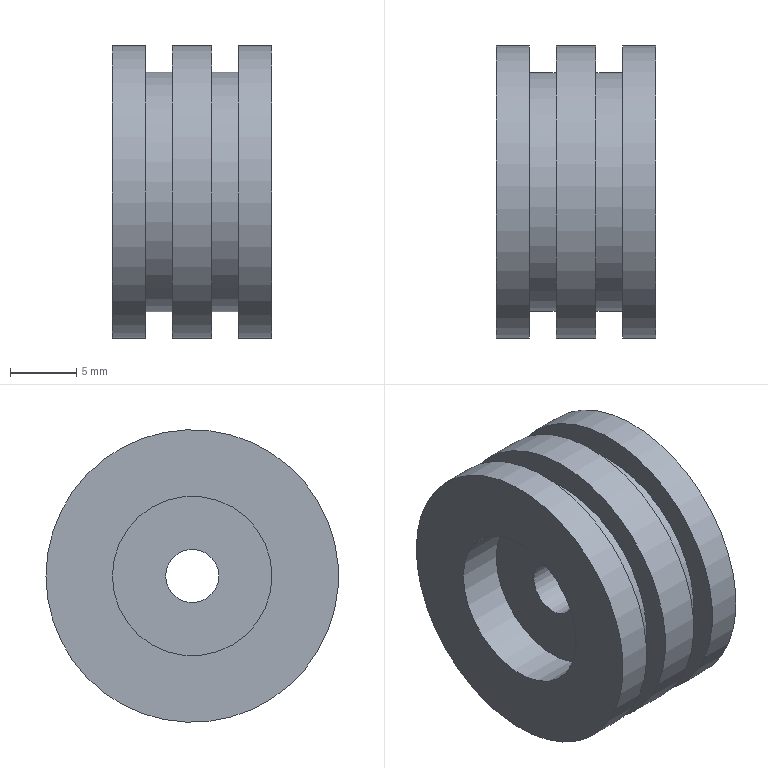Component | NX | PISTON | 1 solid | 16 faces | box 12 x 22 x 22 mm | volume 3525 mm3 | cylinder 8 | plane 8 | commonest cylinder face diameters 22 x3 18 x2 12 x1 6 x1 4 x1
STEP:
#1=CARTESIAN_POINT('',(0.,0.,0.));
#2=DIRECTION('',(0.,0.,1.));
#3=DIRECTION('',(1.,0.,0.));
#4=AXIS2_PLACEMENT_3D('',#1,#2,#3);
#5=CARTESIAN_POINT('',(-114.54,-11.,18.5));
#6=VERTEX_POINT('',#5);
#7=CARTESIAN_POINT('',(-114.54,-22.,18.5));
#8=DIRECTION('',(1.,0.,0.));
#9=DIRECTION('',(0.,1.,0.));
#10=AXIS2_PLACEMENT_3D('',#7,#8,#9);
#11=CIRCLE('',#10,11.);
#12=CARTESIAN_POINT('',(-110.04,-22.,18.5));
#13=DIRECTION('',(-1.,0.,0.));
#14=DIRECTION('',(0.,1.,0.));
#15=AXIS2_PLACEMENT_3D('',#12,#13,#14);
#16=CYLINDRICAL_SURFACE('',#15,11.);
#17=CARTESIAN_POINT('',(6.283,4.5));
#18=DIRECTION('',(-1.,0.));
#19=VECTOR('',#18,1.);
#20=LINE('',#17,#19);
#21=(GEOMETRIC_REPRESENTATION_CONTEXT(2)PARAMETRIC_REPRESENTATION_CONTEXT()REPRESENTATION_CONTEXT('',''));
#22=DEFINITIONAL_REPRESENTATION('',(#20),#21);
#23=PCURVE('',#16,#22);
#24=CARTESIAN_POINT('',(-114.54,-22.,18.5));
#25=DIRECTION('',(1.,0.,0.));
#26=DIRECTION('',(0.,-1.,0.));
#27=AXIS2_PLACEMENT_3D('',#24,#25,#26);
#28=PLANE('',#27);
#29=CARTESIAN_POINT('',(0.,0.));
#30=DIRECTION('',(-1.,0.));
#31=AXIS2_PLACEMENT_2D('',#29,#30);
#32=CIRCLE('',#31,11.);
#33=(GEOMETRIC_REPRESENTATION_CONTEXT(2)PARAMETRIC_REPRESENTATION_CONTEXT()REPRESENTATION_CONTEXT('',''));
#34=DEFINITIONAL_REPRESENTATION('',(#32),#33);
#35=PCURVE('',#28,#34);
#36=SURFACE_CURVE('',#11,(#23,#35),.PCURVE_S1.);
#37=EDGE_CURVE('',#6,#6,#36,.T.);
#38=ORIENTED_EDGE('',*,*,#37,.F.);
#39=CARTESIAN_POINT('',(-117.54,-11.,18.5));
#40=VERTEX_POINT('',#39);
#41=CARTESIAN_POINT('',(-114.54,-11.,18.5));
#42=CARTESIAN_POINT('',(-117.54,-11.,18.5));
#43=B_SPLINE_CURVE_WITH_KNOTS('',1,(#41,#42),.UNSPECIFIED.,.F.,.F.,(2,2),(4.5,7.5),.PIECEWISE_BEZIER_KNOTS.);
#44=CARTESIAN_POINT('',(6.283,0.));
#45=DIRECTION('',(0.,1.));
#46=VECTOR('',#45,1.);
#47=LINE('',#44,#46);
#48=(GEOMETRIC_REPRESENTATION_CONTEXT(2)PARAMETRIC_REPRESENTATION_CONTEXT()REPRESENTATION_CONTEXT('',''));
#49=DEFINITIONAL_REPRESENTATION('',(#47),#48);
#50=PCURVE('',#16,#49);
#51=CARTESIAN_POINT('',(0.,0.));
#52=DIRECTION('',(0.,1.));
#53=VECTOR('',#52,1.);
#54=LINE('',#51,#53);
#55=(GEOMETRIC_REPRESENTATION_CONTEXT(2)PARAMETRIC_REPRESENTATION_CONTEXT()REPRESENTATION_CONTEXT('',''));
#56=DEFINITIONAL_REPRESENTATION('',(#54),#55);
#57=PCURVE('',#16,#56);
#58=SEAM_CURVE('',#43,(#50,#57),.PCURVE_S1.);
#59=EDGE_CURVE('',#6,#40,#58,.T.);
#60=ORIENTED_EDGE('',*,*,#59,.T.);
#61=CARTESIAN_POINT('',(-117.54,-22.,18.5));
#62=DIRECTION('',(-1.,0.,0.));
#63=DIRECTION('',(0.,1.,0.));
#64=AXIS2_PLACEMENT_3D('',#61,#62,#63);
#65=CIRCLE('',#64,11.);
#66=CARTESIAN_POINT('',(0.,7.5));
#67=DIRECTION('',(1.,0.));
#68=VECTOR('',#67,1.);
#69=LINE('',#66,#68);
#70=(GEOMETRIC_REPRESENTATION_CONTEXT(2)PARAMETRIC_REPRESENTATION_CONTEXT()REPRESENTATION_CONTEXT('',''));
#71=DEFINITIONAL_REPRESENTATION('',(#69),#70);
#72=PCURVE('',#16,#71);
#73=CARTESIAN_POINT('',(-117.54,-22.,18.5));
#74=DIRECTION('',(-1.,0.,0.));
#75=DIRECTION('',(0.,1.,0.));
#76=AXIS2_PLACEMENT_3D('',#73,#74,#75);
#77=PLANE('',#76);
#78=CARTESIAN_POINT('',(0.,0.));
#79=DIRECTION('',(1.,0.));
#80=AXIS2_PLACEMENT_2D('',#78,#79);
#81=CIRCLE('',#80,11.);
#82=(GEOMETRIC_REPRESENTATION_CONTEXT(2)PARAMETRIC_REPRESENTATION_CONTEXT()REPRESENTATION_CONTEXT('',''));
#83=DEFINITIONAL_REPRESENTATION('',(#81),#82);
#84=PCURVE('',#77,#83);
#85=SURFACE_CURVE('',#65,(#72,#84),.PCURVE_S1.);
#86=EDGE_CURVE('',#40,#40,#85,.T.);
#87=ORIENTED_EDGE('',*,*,#86,.F.);
#88=ORIENTED_EDGE('',*,*,#59,.F.);
#89=EDGE_LOOP('',(#38,#60,#87,#88));
#90=FACE_BOUND('',#89,.T.);
#91=ADVANCED_FACE('',(#90),#16,.T.);
#92=CARTESIAN_POINT('',(-117.54,-13.,18.5));
#93=VERTEX_POINT('',#92);
#94=CARTESIAN_POINT('',(-117.54,-22.,18.5));
#95=DIRECTION('',(-1.,0.,0.));
#96=DIRECTION('',(0.,1.,0.));
#97=AXIS2_PLACEMENT_3D('',#94,#95,#96);
#98=CIRCLE('',#97,9.);
#99=CARTESIAN_POINT('',(-117.54,-22.,18.5));
#100=DIRECTION('',(-1.,0.,0.));
#101=DIRECTION('',(0.,1.,0.));
#102=AXIS2_PLACEMENT_3D('',#99,#100,#101);
#103=CYLINDRICAL_SURFACE('',#102,9.);
#104=CARTESIAN_POINT('',(0.,0.));
#105=DIRECTION('',(1.,0.));
#106=VECTOR('',#105,1.);
#107=LINE('',#104,#106);
#108=(GEOMETRIC_REPRESENTATION_CONTEXT(2)PARAMETRIC_REPRESENTATION_CONTEXT()REPRESENTATION_CONTEXT('',''));
#109=DEFINITIONAL_REPRESENTATION('',(#107),#108);
#110=PCURVE('',#103,#109);
#111=CARTESIAN_POINT('',(0.,0.));
#112=DIRECTION('',(1.,0.));
#113=AXIS2_PLACEMENT_2D('',#111,#112);
#114=CIRCLE('',#113,9.);
#115=(GEOMETRIC_REPRESENTATION_CONTEXT(2)PARAMETRIC_REPRESENTATION_CONTEXT()REPRESENTATION_CONTEXT('',''));
#116=DEFINITIONAL_REPRESENTATION('',(#114),#115);
#117=PCURVE('',#77,#116);
#118=SURFACE_CURVE('',#98,(#110,#117),.PCURVE_S1.);
#119=EDGE_CURVE('',#93,#93,#118,.T.);
#120=ORIENTED_EDGE('',*,*,#119,.T.);
#121=CARTESIAN_POINT('',(-119.54,-13.,18.5));
#122=VERTEX_POINT('',#121);
#123=CARTESIAN_POINT('',(-117.54,-13.,18.5));
#124=CARTESIAN_POINT('',(-119.54,-13.,18.5));
#125=B_SPLINE_CURVE_WITH_KNOTS('',1,(#123,#124),.UNSPECIFIED.,.F.,.F.,(2,2),(0.,2.),.PIECEWISE_BEZIER_KNOTS.);
#126=CARTESIAN_POINT('',(6.283,0.));
#127=DIRECTION('',(0.,1.));
#128=VECTOR('',#127,1.);
#129=LINE('',#126,#128);
#130=(GEOMETRIC_REPRESENTATION_CONTEXT(2)PARAMETRIC_REPRESENTATION_CONTEXT()REPRESENTATION_CONTEXT('',''));
#131=DEFINITIONAL_REPRESENTATION('',(#129),#130);
#132=PCURVE('',#103,#131);
#133=CARTESIAN_POINT('',(0.,0.));
#134=DIRECTION('',(0.,1.));
#135=VECTOR('',#134,1.);
#136=LINE('',#133,#135);
#137=(GEOMETRIC_REPRESENTATION_CONTEXT(2)PARAMETRIC_REPRESENTATION_CONTEXT()REPRESENTATION_CONTEXT('',''));
#138=DEFINITIONAL_REPRESENTATION('',(#136),#137);
#139=PCURVE('',#103,#138);
#140=SEAM_CURVE('',#125,(#132,#139),.PCURVE_S1.);
#141=EDGE_CURVE('',#93,#122,#140,.T.);
#142=ORIENTED_EDGE('',*,*,#141,.T.);
#143=CARTESIAN_POINT('',(-119.54,-22.,18.5));
#144=DIRECTION('',(-1.,0.,0.));
#145=DIRECTION('',(0.,1.,0.));
#146=AXIS2_PLACEMENT_3D('',#143,#144,#145);
#147=CIRCLE('',#146,9.);
#148=CARTESIAN_POINT('',(0.,2.));
#149=DIRECTION('',(1.,0.));
#150=VECTOR('',#149,1.);
#151=LINE('',#148,#150);
#152=(GEOMETRIC_REPRESENTATION_CONTEXT(2)PARAMETRIC_REPRESENTATION_CONTEXT()REPRESENTATION_CONTEXT('',''));
#153=DEFINITIONAL_REPRESENTATION('',(#151),#152);
#154=PCURVE('',#103,#153);
#155=CARTESIAN_POINT('',(-119.54,-22.,18.5));
#156=DIRECTION('',(-1.,0.,0.));
#157=DIRECTION('',(0.,1.,0.));
#158=AXIS2_PLACEMENT_3D('',#155,#156,#157);
#159=PLANE('',#158);
#160=CARTESIAN_POINT('',(0.,0.));
#161=DIRECTION('',(1.,0.));
#162=AXIS2_PLACEMENT_2D('',#160,#161);
#163=CIRCLE('',#162,9.);
#164=(GEOMETRIC_REPRESENTATION_CONTEXT(2)PARAMETRIC_REPRESENTATION_CONTEXT()REPRESENTATION_CONTEXT('',''));
#165=DEFINITIONAL_REPRESENTATION('',(#163),#164);
#166=PCURVE('',#159,#165);
#167=SURFACE_CURVE('',#147,(#154,#166),.PCURVE_S1.);
#168=EDGE_CURVE('',#122,#122,#167,.T.);
#169=ORIENTED_EDGE('',*,*,#168,.F.);
#170=ORIENTED_EDGE('',*,*,#141,.F.);
#171=EDGE_LOOP('',(#120,#142,#169,#170));
#172=FACE_BOUND('',#171,.T.);
#173=ADVANCED_FACE('',(#172),#103,.T.);
#174=ORIENTED_EDGE('',*,*,#86,.T.);
#175=EDGE_LOOP('',(#174));
#176=FACE_BOUND('',#175,.T.);
#177=ORIENTED_EDGE('',*,*,#119,.F.);
#178=EDGE_LOOP('',(#177));
#179=FACE_BOUND('',#178,.T.);
#180=ADVANCED_FACE('',(#176,#179),#77,.T.);
#181=CARTESIAN_POINT('',(-119.54,-11.,18.5));
#182=VERTEX_POINT('',#181);
#183=CARTESIAN_POINT('',(-119.54,-22.,18.5));
#184=DIRECTION('',(-1.,0.,0.));
#185=DIRECTION('',(0.,1.,0.));
#186=AXIS2_PLACEMENT_3D('',#183,#184,#185);
#187=CIRCLE('',#186,11.);
#188=CARTESIAN_POINT('',(0.,0.));
#189=DIRECTION('',(1.,0.));
#190=AXIS2_PLACEMENT_2D('',#188,#189);
#191=CIRCLE('',#190,11.);
#192=(GEOMETRIC_REPRESENTATION_CONTEXT(2)PARAMETRIC_REPRESENTATION_CONTEXT()REPRESENTATION_CONTEXT('',''));
#193=DEFINITIONAL_REPRESENTATION('',(#191),#192);
#194=PCURVE('',#159,#193);
#195=CARTESIAN_POINT('',(-110.04,-22.,18.5));
#196=DIRECTION('',(-1.,0.,0.));
#197=DIRECTION('',(0.,1.,0.));
#198=AXIS2_PLACEMENT_3D('',#195,#196,#197);
#199=CYLINDRICAL_SURFACE('',#198,11.);
#200=CARTESIAN_POINT('',(0.,9.5));
#201=DIRECTION('',(1.,0.));
#202=VECTOR('',#201,1.);
#203=LINE('',#200,#202);
#204=(GEOMETRIC_REPRESENTATION_CONTEXT(2)PARAMETRIC_REPRESENTATION_CONTEXT()REPRESENTATION_CONTEXT('',''));
#205=DEFINITIONAL_REPRESENTATION('',(#203),#204);
#206=PCURVE('',#199,#205);
#207=SURFACE_CURVE('',#187,(#194,#206),.PCURVE_S1.);
#208=EDGE_CURVE('',#182,#182,#207,.T.);
#209=ORIENTED_EDGE('',*,*,#208,.F.);
#210=EDGE_LOOP('',(#209));
#211=FACE_BOUND('',#210,.T.);
#212=ORIENTED_EDGE('',*,*,#168,.T.);
#213=EDGE_LOOP('',(#212));
#214=FACE_BOUND('',#213,.T.);
#215=ADVANCED_FACE('',(#211,#214),#159,.F.);
#216=CARTESIAN_POINT('',(-122.04,-16.,18.5));
#217=VERTEX_POINT('',#216);
#218=CARTESIAN_POINT('',(-122.04,-22.,18.5));
#219=DIRECTION('',(1.,0.,0.));
#220=DIRECTION('',(0.,1.,0.));
#221=AXIS2_PLACEMENT_3D('',#218,#219,#220);
#222=CIRCLE('',#221,6.);
#223=CARTESIAN_POINT('',(-122.04,-22.,18.5));
#224=DIRECTION('',(-1.,0.,0.));
#225=DIRECTION('',(0.,1.,0.));
#226=AXIS2_PLACEMENT_3D('',#223,#224,#225);
#227=PLANE('',#226);
#228=CARTESIAN_POINT('',(6.,0.));
#229=CARTESIAN_POINT('',(6.,-10.392));
#230=CARTESIAN_POINT('',(-3.,-5.196));
#231=CARTESIAN_POINT('',(-12.,-0.));
#232=CARTESIAN_POINT('',(-3.,5.196));
#233=CARTESIAN_POINT('',(6.,10.392));
#234=CARTESIAN_POINT('',(6.,0.));
#235=(BOUNDED_CURVE()B_SPLINE_CURVE(2,(#228,#229,#230,#231,#232,#233,#234),.UNSPECIFIED.,.T.,.F.)B_SPLINE_CURVE_WITH_KNOTS((1,2,2,2,2,1),(-2.094,0.,2.094,4.189,6.283,8.378),.UNSPECIFIED.)CURVE()GEOMETRIC_REPRESENTATION_ITEM()RATIONAL_B_SPLINE_CURVE((1.,0.5,1.,0.5,1.,0.5,1.))REPRESENTATION_ITEM(''));
#236=(GEOMETRIC_REPRESENTATION_CONTEXT(2)PARAMETRIC_REPRESENTATION_CONTEXT()REPRESENTATION_CONTEXT('',''));
#237=DEFINITIONAL_REPRESENTATION('',(#235),#236);
#238=PCURVE('',#227,#237);
#239=CARTESIAN_POINT('',(-118.54,-22.,18.5));
#240=DIRECTION('',(-1.,0.,0.));
#241=DIRECTION('',(0.,1.,0.));
#242=AXIS2_PLACEMENT_3D('',#239,#240,#241);
#243=CYLINDRICAL_SURFACE('',#242,6.);
#244=CARTESIAN_POINT('',(6.283,3.5));
#245=DIRECTION('',(-1.,0.));
#246=VECTOR('',#245,1.);
#247=LINE('',#244,#246);
#248=(GEOMETRIC_REPRESENTATION_CONTEXT(2)PARAMETRIC_REPRESENTATION_CONTEXT()REPRESENTATION_CONTEXT('',''));
#249=DEFINITIONAL_REPRESENTATION('',(#247),#248);
#250=PCURVE('',#243,#249);
#251=SURFACE_CURVE('',#222,(#238,#250),.PCURVE_S1.);
#252=EDGE_CURVE('',#217,#217,#251,.T.);
#253=ORIENTED_EDGE('',*,*,#252,.T.);
#254=EDGE_LOOP('',(#253));
#255=FACE_BOUND('',#254,.T.);
#256=CARTESIAN_POINT('',(-122.04,-11.,18.5));
#257=VERTEX_POINT('',#256);
#258=CARTESIAN_POINT('',(-122.04,-22.,18.5));
#259=DIRECTION('',(1.,0.,0.));
#260=DIRECTION('',(0.,1.,0.));
#261=AXIS2_PLACEMENT_3D('',#258,#259,#260);
#262=CIRCLE('',#261,11.);
#263=CARTESIAN_POINT('',(11.,0.));
#264=CARTESIAN_POINT('',(11.,-19.053));
#265=CARTESIAN_POINT('',(-5.5,-9.526));
#266=CARTESIAN_POINT('',(-22.,-0.));
#267=CARTESIAN_POINT('',(-5.5,9.526));
#268=CARTESIAN_POINT('',(11.,19.053));
#269=CARTESIAN_POINT('',(11.,0.));
#270=(BOUNDED_CURVE()B_SPLINE_CURVE(2,(#263,#264,#265,#266,#267,#268,#269),.UNSPECIFIED.,.T.,.F.)B_SPLINE_CURVE_WITH_KNOTS((1,2,2,2,2,1),(-2.094,0.,2.094,4.189,6.283,8.378),.UNSPECIFIED.)CURVE()GEOMETRIC_REPRESENTATION_ITEM()RATIONAL_B_SPLINE_CURVE((1.,0.5,1.,0.5,1.,0.5,1.))REPRESENTATION_ITEM(''));
#271=(GEOMETRIC_REPRESENTATION_CONTEXT(2)PARAMETRIC_REPRESENTATION_CONTEXT()REPRESENTATION_CONTEXT('',''));
#272=DEFINITIONAL_REPRESENTATION('',(#270),#271);
#273=PCURVE('',#227,#272);
#274=CARTESIAN_POINT('',(6.283,12.));
#275=DIRECTION('',(-1.,0.));
#276=VECTOR('',#275,1.);
#277=LINE('',#274,#276);
#278=(GEOMETRIC_REPRESENTATION_CONTEXT(2)PARAMETRIC_REPRESENTATION_CONTEXT()REPRESENTATION_CONTEXT('',''));
#279=DEFINITIONAL_REPRESENTATION('',(#277),#278);
#280=PCURVE('',#199,#279);
#281=SURFACE_CURVE('',#262,(#273,#280),.PCURVE_S1.);
#282=EDGE_CURVE('',#257,#257,#281,.T.);
#283=ORIENTED_EDGE('',*,*,#282,.F.);
#284=EDGE_LOOP('',(#283));
#285=FACE_BOUND('',#284,.T.);
#286=ADVANCED_FACE('',(#255,#285),#227,.T.);
#287=ORIENTED_EDGE('',*,*,#282,.T.);
#288=CARTESIAN_POINT('',(-119.54,-11.,18.5));
#289=CARTESIAN_POINT('',(-122.04,-11.,18.5));
#290=B_SPLINE_CURVE_WITH_KNOTS('',1,(#288,#289),.UNSPECIFIED.,.F.,.F.,(2,2),(9.5,12.),.PIECEWISE_BEZIER_KNOTS.);
#291=CARTESIAN_POINT('',(0.,0.));
#292=DIRECTION('',(0.,1.));
#293=VECTOR('',#292,1.);
#294=LINE('',#291,#293);
#295=(GEOMETRIC_REPRESENTATION_CONTEXT(2)PARAMETRIC_REPRESENTATION_CONTEXT()REPRESENTATION_CONTEXT('',''));
#296=DEFINITIONAL_REPRESENTATION('',(#294),#295);
#297=PCURVE('',#199,#296);
#298=CARTESIAN_POINT('',(6.283,0.));
#299=DIRECTION('',(0.,1.));
#300=VECTOR('',#299,1.);
#301=LINE('',#298,#300);
#302=(GEOMETRIC_REPRESENTATION_CONTEXT(2)PARAMETRIC_REPRESENTATION_CONTEXT()REPRESENTATION_CONTEXT('',''));
#303=DEFINITIONAL_REPRESENTATION('',(#301),#302);
#304=PCURVE('',#199,#303);
#305=SEAM_CURVE('',#290,(#297,#304),.PCURVE_S1.);
#306=EDGE_CURVE('',#182,#257,#305,.T.);
#307=ORIENTED_EDGE('',*,*,#306,.F.);
#308=ORIENTED_EDGE('',*,*,#208,.T.);
#309=ORIENTED_EDGE('',*,*,#306,.T.);
#310=EDGE_LOOP('',(#287,#307,#308,#309));
#311=FACE_BOUND('',#310,.T.);
#312=ADVANCED_FACE('',(#311),#199,.T.);
#313=CARTESIAN_POINT('',(-114.54,-13.,18.5));
#314=VERTEX_POINT('',#313);
#315=CARTESIAN_POINT('',(-114.54,-22.,18.5));
#316=DIRECTION('',(1.,0.,0.));
#317=DIRECTION('',(0.,1.,0.));
#318=AXIS2_PLACEMENT_3D('',#315,#316,#317);
#319=CIRCLE('',#318,9.);
#320=CARTESIAN_POINT('',(-114.54,-22.,18.5));
#321=DIRECTION('',(1.,0.,0.));
#322=DIRECTION('',(0.,-1.,0.));
#323=AXIS2_PLACEMENT_3D('',#320,#321,#322);
#324=CYLINDRICAL_SURFACE('',#323,9.);
#325=CARTESIAN_POINT('',(3.142,0.));
#326=DIRECTION('',(1.,0.));
#327=VECTOR('',#326,1.);
#328=LINE('',#325,#327);
#329=(GEOMETRIC_REPRESENTATION_CONTEXT(2)PARAMETRIC_REPRESENTATION_CONTEXT()REPRESENTATION_CONTEXT('',''));
#330=DEFINITIONAL_REPRESENTATION('',(#328),#329);
#331=PCURVE('',#324,#330);
#332=CARTESIAN_POINT('',(0.,0.));
#333=DIRECTION('',(-1.,0.));
#334=AXIS2_PLACEMENT_2D('',#332,#333);
#335=CIRCLE('',#334,9.);
#336=(GEOMETRIC_REPRESENTATION_CONTEXT(2)PARAMETRIC_REPRESENTATION_CONTEXT()REPRESENTATION_CONTEXT('',''));
#337=DEFINITIONAL_REPRESENTATION('',(#335),#336);
#338=PCURVE('',#28,#337);
#339=SURFACE_CURVE('',#319,(#331,#338),.PCURVE_S1.);
#340=EDGE_CURVE('',#314,#314,#339,.T.);
#341=ORIENTED_EDGE('',*,*,#340,.T.);
#342=CARTESIAN_POINT('',(-112.54,-13.,18.5));
#343=VERTEX_POINT('',#342);
#344=CARTESIAN_POINT('',(-114.54,-13.,18.5));
#345=CARTESIAN_POINT('',(-112.54,-13.,18.5));
#346=B_SPLINE_CURVE_WITH_KNOTS('',1,(#344,#345),.UNSPECIFIED.,.F.,.F.,(2,2),(0.,2.),.PIECEWISE_BEZIER_KNOTS.);
#347=CARTESIAN_POINT('',(9.425,0.));
#348=DIRECTION('',(0.,1.));
#349=VECTOR('',#348,1.);
#350=LINE('',#347,#349);
#351=(GEOMETRIC_REPRESENTATION_CONTEXT(2)PARAMETRIC_REPRESENTATION_CONTEXT()REPRESENTATION_CONTEXT('',''));
#352=DEFINITIONAL_REPRESENTATION('',(#350),#351);
#353=PCURVE('',#324,#352);
#354=CARTESIAN_POINT('',(3.142,0.));
#355=DIRECTION('',(0.,1.));
#356=VECTOR('',#355,1.);
#357=LINE('',#354,#356);
#358=(GEOMETRIC_REPRESENTATION_CONTEXT(2)PARAMETRIC_REPRESENTATION_CONTEXT()REPRESENTATION_CONTEXT('',''));
#359=DEFINITIONAL_REPRESENTATION('',(#357),#358);
#360=PCURVE('',#324,#359);
#361=SEAM_CURVE('',#346,(#353,#360),.PCURVE_S1.);
#362=EDGE_CURVE('',#314,#343,#361,.T.);
#363=ORIENTED_EDGE('',*,*,#362,.T.);
#364=CARTESIAN_POINT('',(-112.54,-22.,18.5));
#365=DIRECTION('',(1.,0.,0.));
#366=DIRECTION('',(0.,1.,0.));
#367=AXIS2_PLACEMENT_3D('',#364,#365,#366);
#368=CIRCLE('',#367,9.);
#369=CARTESIAN_POINT('',(3.142,2.));
#370=DIRECTION('',(1.,0.));
#371=VECTOR('',#370,1.);
#372=LINE('',#369,#371);
#373=(GEOMETRIC_REPRESENTATION_CONTEXT(2)PARAMETRIC_REPRESENTATION_CONTEXT()REPRESENTATION_CONTEXT('',''));
#374=DEFINITIONAL_REPRESENTATION('',(#372),#373);
#375=PCURVE('',#324,#374);
#376=CARTESIAN_POINT('',(-112.54,-22.,18.5));
#377=DIRECTION('',(1.,0.,0.));
#378=DIRECTION('',(0.,-1.,0.));
#379=AXIS2_PLACEMENT_3D('',#376,#377,#378);
#380=PLANE('',#379);
#381=CARTESIAN_POINT('',(0.,0.));
#382=DIRECTION('',(-1.,0.));
#383=AXIS2_PLACEMENT_2D('',#381,#382);
#384=CIRCLE('',#383,9.);
#385=(GEOMETRIC_REPRESENTATION_CONTEXT(2)PARAMETRIC_REPRESENTATION_CONTEXT()REPRESENTATION_CONTEXT('',''));
#386=DEFINITIONAL_REPRESENTATION('',(#384),#385);
#387=PCURVE('',#380,#386);
#388=SURFACE_CURVE('',#368,(#375,#387),.PCURVE_S1.);
#389=EDGE_CURVE('',#343,#343,#388,.T.);
#390=ORIENTED_EDGE('',*,*,#389,.F.);
#391=ORIENTED_EDGE('',*,*,#362,.F.);
#392=EDGE_LOOP('',(#341,#363,#390,#391));
#393=FACE_BOUND('',#392,.T.);
#394=ADVANCED_FACE('',(#393),#324,.T.);
#395=ORIENTED_EDGE('',*,*,#37,.T.);
#396=EDGE_LOOP('',(#395));
#397=FACE_BOUND('',#396,.T.);
#398=ORIENTED_EDGE('',*,*,#340,.F.);
#399=EDGE_LOOP('',(#398));
#400=FACE_BOUND('',#399,.T.);
#401=ADVANCED_FACE('',(#397,#400),#28,.T.);
#402=CARTESIAN_POINT('',(-112.54,-11.,18.5));
#403=VERTEX_POINT('',#402);
#404=CARTESIAN_POINT('',(-112.54,-22.,18.5));
#405=DIRECTION('',(1.,0.,0.));
#406=DIRECTION('',(0.,1.,0.));
#407=AXIS2_PLACEMENT_3D('',#404,#405,#406);
#408=CIRCLE('',#407,11.);
#409=CARTESIAN_POINT('',(0.,0.));
#410=DIRECTION('',(-1.,0.));
#411=AXIS2_PLACEMENT_2D('',#409,#410);
#412=CIRCLE('',#411,11.);
#413=(GEOMETRIC_REPRESENTATION_CONTEXT(2)PARAMETRIC_REPRESENTATION_CONTEXT()REPRESENTATION_CONTEXT('',''));
#414=DEFINITIONAL_REPRESENTATION('',(#412),#413);
#415=PCURVE('',#380,#414);
#416=CARTESIAN_POINT('',(-110.04,-22.,18.5));
#417=DIRECTION('',(-1.,0.,0.));
#418=DIRECTION('',(0.,1.,0.));
#419=AXIS2_PLACEMENT_3D('',#416,#417,#418);
#420=CYLINDRICAL_SURFACE('',#419,11.);
#421=CARTESIAN_POINT('',(6.283,2.5));
#422=DIRECTION('',(-1.,0.));
#423=VECTOR('',#422,1.);
#424=LINE('',#421,#423);
#425=(GEOMETRIC_REPRESENTATION_CONTEXT(2)PARAMETRIC_REPRESENTATION_CONTEXT()REPRESENTATION_CONTEXT('',''));
#426=DEFINITIONAL_REPRESENTATION('',(#424),#425);
#427=PCURVE('',#420,#426);
#428=SURFACE_CURVE('',#408,(#415,#427),.PCURVE_S1.);
#429=EDGE_CURVE('',#403,#403,#428,.T.);
#430=ORIENTED_EDGE('',*,*,#429,.F.);
#431=EDGE_LOOP('',(#430));
#432=FACE_BOUND('',#431,.T.);
#433=ORIENTED_EDGE('',*,*,#389,.T.);
#434=EDGE_LOOP('',(#433));
#435=FACE_BOUND('',#434,.T.);
#436=ADVANCED_FACE('',(#432,#435),#380,.F.);
#437=CARTESIAN_POINT('',(-110.04,-19.,18.5));
#438=VERTEX_POINT('',#437);
#439=CARTESIAN_POINT('',(-110.04,-22.,18.5));
#440=DIRECTION('',(-1.,0.,0.));
#441=DIRECTION('',(0.,1.,0.));
#442=AXIS2_PLACEMENT_3D('',#439,#440,#441);
#443=CIRCLE('',#442,3.);
#444=CARTESIAN_POINT('',(-110.04,-22.,18.5));
#445=DIRECTION('',(1.,0.,0.));
#446=DIRECTION('',(0.,-1.,0.));
#447=AXIS2_PLACEMENT_3D('',#444,#445,#446);
#448=PLANE('',#447);
#449=CARTESIAN_POINT('',(-3.,0.));
#450=CARTESIAN_POINT('',(-3.,5.196));
#451=CARTESIAN_POINT('',(1.5,2.598));
#452=CARTESIAN_POINT('',(6.,0.));
#453=CARTESIAN_POINT('',(1.5,-2.598));
#454=CARTESIAN_POINT('',(-3.,-5.196));
#455=CARTESIAN_POINT('',(-3.,0.));
#456=(BOUNDED_CURVE()B_SPLINE_CURVE(2,(#449,#450,#451,#452,#453,#454,#455),.UNSPECIFIED.,.T.,.F.)B_SPLINE_CURVE_WITH_KNOTS((1,2,2,2,2,1),(-2.094,0.,2.094,4.189,6.283,8.378),.UNSPECIFIED.)CURVE()GEOMETRIC_REPRESENTATION_ITEM()RATIONAL_B_SPLINE_CURVE((1.,0.5,1.,0.5,1.,0.5,1.))REPRESENTATION_ITEM(''));
#457=(GEOMETRIC_REPRESENTATION_CONTEXT(2)PARAMETRIC_REPRESENTATION_CONTEXT()REPRESENTATION_CONTEXT('',''));
#458=DEFINITIONAL_REPRESENTATION('',(#456),#457);
#459=PCURVE('',#448,#458);
#460=CARTESIAN_POINT('',(-112.04,-22.,18.5));
#461=DIRECTION('',(1.,0.,0.));
#462=DIRECTION('',(0.,-1.,0.));
#463=AXIS2_PLACEMENT_3D('',#460,#461,#462);
#464=CYLINDRICAL_SURFACE('',#463,3.);
#465=CARTESIAN_POINT('',(9.425,2.));
#466=DIRECTION('',(-1.,0.));
#467=VECTOR('',#466,1.);
#468=LINE('',#465,#467);
#469=(GEOMETRIC_REPRESENTATION_CONTEXT(2)PARAMETRIC_REPRESENTATION_CONTEXT()REPRESENTATION_CONTEXT('',''));
#470=DEFINITIONAL_REPRESENTATION('',(#468),#469);
#471=PCURVE('',#464,#470);
#472=SURFACE_CURVE('',#443,(#459,#471),.PCURVE_S1.);
#473=EDGE_CURVE('',#438,#438,#472,.T.);
#474=ORIENTED_EDGE('',*,*,#473,.T.);
#475=EDGE_LOOP('',(#474));
#476=FACE_BOUND('',#475,.T.);
#477=CARTESIAN_POINT('',(-110.04,-11.,18.5));
#478=VERTEX_POINT('',#477);
#479=CARTESIAN_POINT('',(-110.04,-22.,18.5));
#480=DIRECTION('',(-1.,0.,0.));
#481=DIRECTION('',(0.,1.,0.));
#482=AXIS2_PLACEMENT_3D('',#479,#480,#481);
#483=CIRCLE('',#482,11.);
#484=CARTESIAN_POINT('',(-11.,0.));
#485=CARTESIAN_POINT('',(-11.,19.053));
#486=CARTESIAN_POINT('',(5.5,9.526));
#487=CARTESIAN_POINT('',(22.,0.));
#488=CARTESIAN_POINT('',(5.5,-9.526));
#489=CARTESIAN_POINT('',(-11.,-19.053));
#490=CARTESIAN_POINT('',(-11.,0.));
#491=(BOUNDED_CURVE()B_SPLINE_CURVE(2,(#484,#485,#486,#487,#488,#489,#490),.UNSPECIFIED.,.T.,.F.)B_SPLINE_CURVE_WITH_KNOTS((1,2,2,2,2,1),(-2.094,0.,2.094,4.189,6.283,8.378),.UNSPECIFIED.)CURVE()GEOMETRIC_REPRESENTATION_ITEM()RATIONAL_B_SPLINE_CURVE((1.,0.5,1.,0.5,1.,0.5,1.))REPRESENTATION_ITEM(''));
#492=(GEOMETRIC_REPRESENTATION_CONTEXT(2)PARAMETRIC_REPRESENTATION_CONTEXT()REPRESENTATION_CONTEXT('',''));
#493=DEFINITIONAL_REPRESENTATION('',(#491),#492);
#494=PCURVE('',#448,#493);
#495=CARTESIAN_POINT('',(0.,0.));
#496=DIRECTION('',(1.,0.));
#497=VECTOR('',#496,1.);
#498=LINE('',#495,#497);
#499=(GEOMETRIC_REPRESENTATION_CONTEXT(2)PARAMETRIC_REPRESENTATION_CONTEXT()REPRESENTATION_CONTEXT('',''));
#500=DEFINITIONAL_REPRESENTATION('',(#498),#499);
#501=PCURVE('',#420,#500);
#502=SURFACE_CURVE('',#483,(#494,#501),.PCURVE_S1.);
#503=EDGE_CURVE('',#478,#478,#502,.T.);
#504=ORIENTED_EDGE('',*,*,#503,.F.);
#505=EDGE_LOOP('',(#504));
#506=FACE_BOUND('',#505,.T.);
#507=ADVANCED_FACE('',(#476,#506),#448,.T.);
#508=ORIENTED_EDGE('',*,*,#503,.T.);
#509=CARTESIAN_POINT('',(-110.04,-11.,18.5));
#510=CARTESIAN_POINT('',(-112.54,-11.,18.5));
#511=B_SPLINE_CURVE_WITH_KNOTS('',1,(#509,#510),.UNSPECIFIED.,.F.,.F.,(2,2),(0.,2.5),.PIECEWISE_BEZIER_KNOTS.);
#512=CARTESIAN_POINT('',(6.283,0.));
#513=DIRECTION('',(0.,1.));
#514=VECTOR('',#513,1.);
#515=LINE('',#512,#514);
#516=(GEOMETRIC_REPRESENTATION_CONTEXT(2)PARAMETRIC_REPRESENTATION_CONTEXT()REPRESENTATION_CONTEXT('',''));
#517=DEFINITIONAL_REPRESENTATION('',(#515),#516);
#518=PCURVE('',#420,#517);
#519=CARTESIAN_POINT('',(0.,0.));
#520=DIRECTION('',(0.,1.));
#521=VECTOR('',#520,1.);
#522=LINE('',#519,#521);
#523=(GEOMETRIC_REPRESENTATION_CONTEXT(2)PARAMETRIC_REPRESENTATION_CONTEXT()REPRESENTATION_CONTEXT('',''));
#524=DEFINITIONAL_REPRESENTATION('',(#522),#523);
#525=PCURVE('',#420,#524);
#526=SEAM_CURVE('',#511,(#518,#525),.PCURVE_S1.);
#527=EDGE_CURVE('',#478,#403,#526,.T.);
#528=ORIENTED_EDGE('',*,*,#527,.T.);
#529=ORIENTED_EDGE('',*,*,#429,.T.);
#530=ORIENTED_EDGE('',*,*,#527,.F.);
#531=EDGE_LOOP('',(#508,#528,#529,#530));
#532=FACE_BOUND('',#531,.T.);
#533=ADVANCED_FACE('',(#532),#420,.T.);
#534=CARTESIAN_POINT('',(-118.54,-16.,18.5));
#535=VERTEX_POINT('',#534);
#536=CARTESIAN_POINT('',(-118.54,-22.,18.5));
#537=DIRECTION('',(-1.,0.,0.));
#538=DIRECTION('',(0.,1.,0.));
#539=AXIS2_PLACEMENT_3D('',#536,#537,#538);
#540=CIRCLE('',#539,6.);
#541=CARTESIAN_POINT('',(0.,0.));
#542=DIRECTION('',(1.,0.));
#543=VECTOR('',#542,1.);
#544=LINE('',#541,#543);
#545=(GEOMETRIC_REPRESENTATION_CONTEXT(2)PARAMETRIC_REPRESENTATION_CONTEXT()REPRESENTATION_CONTEXT('',''));
#546=DEFINITIONAL_REPRESENTATION('',(#544),#545);
#547=PCURVE('',#243,#546);
#548=CARTESIAN_POINT('',(-118.54,-22.,18.5));
#549=DIRECTION('',(1.,0.,0.));
#550=DIRECTION('',(0.,-1.,0.));
#551=AXIS2_PLACEMENT_3D('',#548,#549,#550);
#552=PLANE('',#551);
#553=CARTESIAN_POINT('',(-6.,0.));
#554=CARTESIAN_POINT('',(-6.,10.392));
#555=CARTESIAN_POINT('',(3.,5.196));
#556=CARTESIAN_POINT('',(12.,0.));
#557=CARTESIAN_POINT('',(3.,-5.196));
#558=CARTESIAN_POINT('',(-6.,-10.392));
#559=CARTESIAN_POINT('',(-6.,0.));
#560=(BOUNDED_CURVE()B_SPLINE_CURVE(2,(#553,#554,#555,#556,#557,#558,#559),.UNSPECIFIED.,.T.,.F.)B_SPLINE_CURVE_WITH_KNOTS((1,2,2,2,2,1),(-2.094,0.,2.094,4.189,6.283,8.378),.UNSPECIFIED.)CURVE()GEOMETRIC_REPRESENTATION_ITEM()RATIONAL_B_SPLINE_CURVE((1.,0.5,1.,0.5,1.,0.5,1.))REPRESENTATION_ITEM(''));
#561=(GEOMETRIC_REPRESENTATION_CONTEXT(2)PARAMETRIC_REPRESENTATION_CONTEXT()REPRESENTATION_CONTEXT('',''));
#562=DEFINITIONAL_REPRESENTATION('',(#560),#561);
#563=PCURVE('',#552,#562);
#564=SURFACE_CURVE('',#540,(#547,#563),.PCURVE_S1.);
#565=EDGE_CURVE('',#535,#535,#564,.T.);
#566=ORIENTED_EDGE('',*,*,#565,.T.);
#567=CARTESIAN_POINT('',(-118.54,-16.,18.5));
#568=CARTESIAN_POINT('',(-122.04,-16.,18.5));
#569=B_SPLINE_CURVE_WITH_KNOTS('',1,(#567,#568),.UNSPECIFIED.,.F.,.F.,(2,2),(0.,3.5),.PIECEWISE_BEZIER_KNOTS.);
#570=CARTESIAN_POINT('',(6.283,0.));
#571=DIRECTION('',(0.,1.));
#572=VECTOR('',#571,1.);
#573=LINE('',#570,#572);
#574=(GEOMETRIC_REPRESENTATION_CONTEXT(2)PARAMETRIC_REPRESENTATION_CONTEXT()REPRESENTATION_CONTEXT('',''));
#575=DEFINITIONAL_REPRESENTATION('',(#573),#574);
#576=PCURVE('',#243,#575);
#577=CARTESIAN_POINT('',(0.,0.));
#578=DIRECTION('',(0.,1.));
#579=VECTOR('',#578,1.);
#580=LINE('',#577,#579);
#581=(GEOMETRIC_REPRESENTATION_CONTEXT(2)PARAMETRIC_REPRESENTATION_CONTEXT()REPRESENTATION_CONTEXT('',''));
#582=DEFINITIONAL_REPRESENTATION('',(#580),#581);
#583=PCURVE('',#243,#582);
#584=SEAM_CURVE('',#569,(#576,#583),.PCURVE_S1.);
#585=EDGE_CURVE('',#535,#217,#584,.T.);
#586=ORIENTED_EDGE('',*,*,#585,.T.);
#587=ORIENTED_EDGE('',*,*,#252,.T.);
#588=ORIENTED_EDGE('',*,*,#585,.F.);
#589=EDGE_LOOP('',(#566,#586,#587,#588));
#590=FACE_BOUND('',#589,.F.);
#591=ADVANCED_FACE('',(#590),#243,.F.);
#592=CARTESIAN_POINT('',(-118.54,-24.,18.5));
#593=VERTEX_POINT('',#592);
#594=CARTESIAN_POINT('',(-118.54,-22.,18.5));
#595=DIRECTION('',(-1.,0.,0.));
#596=DIRECTION('',(0.,-1.,0.));
#597=AXIS2_PLACEMENT_3D('',#594,#595,#596);
#598=CIRCLE('',#597,2.);
#599=CARTESIAN_POINT('',(2.,0.));
#600=CARTESIAN_POINT('',(2.,-3.464));
#601=CARTESIAN_POINT('',(-1.,-1.732));
#602=CARTESIAN_POINT('',(-4.,-0.));
#603=CARTESIAN_POINT('',(-1.,1.732));
#604=CARTESIAN_POINT('',(2.,3.464));
#605=CARTESIAN_POINT('',(2.,0.));
#606=(BOUNDED_CURVE()B_SPLINE_CURVE(2,(#599,#600,#601,#602,#603,#604,#605),.UNSPECIFIED.,.T.,.F.)B_SPLINE_CURVE_WITH_KNOTS((1,2,2,2,2,1),(-2.094,0.,2.094,4.189,6.283,8.378),.UNSPECIFIED.)CURVE()GEOMETRIC_REPRESENTATION_ITEM()RATIONAL_B_SPLINE_CURVE((1.,0.5,1.,0.5,1.,0.5,1.))REPRESENTATION_ITEM(''));
#607=(GEOMETRIC_REPRESENTATION_CONTEXT(2)PARAMETRIC_REPRESENTATION_CONTEXT()REPRESENTATION_CONTEXT('',''));
#608=DEFINITIONAL_REPRESENTATION('',(#606),#607);
#609=PCURVE('',#552,#608);
#610=CARTESIAN_POINT('',(-132.04,-22.,18.5));
#611=DIRECTION('',(1.,0.,0.));
#612=DIRECTION('',(0.,-1.,0.));
#613=AXIS2_PLACEMENT_3D('',#610,#611,#612);
#614=CYLINDRICAL_SURFACE('',#613,2.);
#615=CARTESIAN_POINT('',(6.283,13.5));
#616=DIRECTION('',(-1.,0.));
#617=VECTOR('',#616,1.);
#618=LINE('',#615,#617);
#619=(GEOMETRIC_REPRESENTATION_CONTEXT(2)PARAMETRIC_REPRESENTATION_CONTEXT()REPRESENTATION_CONTEXT('',''));
#620=DEFINITIONAL_REPRESENTATION('',(#618),#619);
#621=PCURVE('',#614,#620);
#622=SURFACE_CURVE('',#598,(#609,#621),.PCURVE_S1.);
#623=EDGE_CURVE('',#593,#593,#622,.T.);
#624=ORIENTED_EDGE('',*,*,#623,.F.);
#625=EDGE_LOOP('',(#624));
#626=FACE_BOUND('',#625,.T.);
#627=ORIENTED_EDGE('',*,*,#565,.T.);
#628=EDGE_LOOP('',(#627));
#629=FACE_BOUND('',#628,.T.);
#630=ADVANCED_FACE('',(#626,#629),#552,.F.);
#631=CARTESIAN_POINT('',(-112.04,-19.,18.5));
#632=VERTEX_POINT('',#631);
#633=CARTESIAN_POINT('',(-112.04,-22.,18.5));
#634=DIRECTION('',(1.,0.,0.));
#635=DIRECTION('',(0.,1.,0.));
#636=AXIS2_PLACEMENT_3D('',#633,#634,#635);
#637=CIRCLE('',#636,3.);
#638=CARTESIAN_POINT('',(3.142,0.));
#639=DIRECTION('',(1.,0.));
#640=VECTOR('',#639,1.);
#641=LINE('',#638,#640);
#642=(GEOMETRIC_REPRESENTATION_CONTEXT(2)PARAMETRIC_REPRESENTATION_CONTEXT()REPRESENTATION_CONTEXT('',''));
#643=DEFINITIONAL_REPRESENTATION('',(#641),#642);
#644=PCURVE('',#464,#643);
#645=CARTESIAN_POINT('',(-112.04,-22.,18.5));
#646=DIRECTION('',(-1.,0.,0.));
#647=DIRECTION('',(0.,1.,0.));
#648=AXIS2_PLACEMENT_3D('',#645,#646,#647);
#649=PLANE('',#648);
#650=CARTESIAN_POINT('',(3.,0.));
#651=CARTESIAN_POINT('',(3.,-5.196));
#652=CARTESIAN_POINT('',(-1.5,-2.598));
#653=CARTESIAN_POINT('',(-6.,-0.));
#654=CARTESIAN_POINT('',(-1.5,2.598));
#655=CARTESIAN_POINT('',(3.,5.196));
#656=CARTESIAN_POINT('',(3.,0.));
#657=(BOUNDED_CURVE()B_SPLINE_CURVE(2,(#650,#651,#652,#653,#654,#655,#656),.UNSPECIFIED.,.T.,.F.)B_SPLINE_CURVE_WITH_KNOTS((1,2,2,2,2,1),(-2.094,0.,2.094,4.189,6.283,8.378),.UNSPECIFIED.)CURVE()GEOMETRIC_REPRESENTATION_ITEM()RATIONAL_B_SPLINE_CURVE((1.,0.5,1.,0.5,1.,0.5,1.))REPRESENTATION_ITEM(''));
#658=(GEOMETRIC_REPRESENTATION_CONTEXT(2)PARAMETRIC_REPRESENTATION_CONTEXT()REPRESENTATION_CONTEXT('',''));
#659=DEFINITIONAL_REPRESENTATION('',(#657),#658);
#660=PCURVE('',#649,#659);
#661=SURFACE_CURVE('',#637,(#644,#660),.PCURVE_S1.);
#662=EDGE_CURVE('',#632,#632,#661,.T.);
#663=ORIENTED_EDGE('',*,*,#662,.T.);
#664=CARTESIAN_POINT('',(-112.04,-19.,18.5));
#665=CARTESIAN_POINT('',(-110.04,-19.,18.5));
#666=B_SPLINE_CURVE_WITH_KNOTS('',1,(#664,#665),.UNSPECIFIED.,.F.,.F.,(2,2),(0.,2.),.PIECEWISE_BEZIER_KNOTS.);
#667=CARTESIAN_POINT('',(9.425,0.));
#668=DIRECTION('',(0.,1.));
#669=VECTOR('',#668,1.);
#670=LINE('',#667,#669);
#671=(GEOMETRIC_REPRESENTATION_CONTEXT(2)PARAMETRIC_REPRESENTATION_CONTEXT()REPRESENTATION_CONTEXT('',''));
#672=DEFINITIONAL_REPRESENTATION('',(#670),#671);
#673=PCURVE('',#464,#672);
#674=CARTESIAN_POINT('',(3.142,0.));
#675=DIRECTION('',(0.,1.));
#676=VECTOR('',#675,1.);
#677=LINE('',#674,#676);
#678=(GEOMETRIC_REPRESENTATION_CONTEXT(2)PARAMETRIC_REPRESENTATION_CONTEXT()REPRESENTATION_CONTEXT('',''));
#679=DEFINITIONAL_REPRESENTATION('',(#677),#678);
#680=PCURVE('',#464,#679);
#681=SEAM_CURVE('',#666,(#673,#680),.PCURVE_S1.);
#682=EDGE_CURVE('',#632,#438,#681,.T.);
#683=ORIENTED_EDGE('',*,*,#682,.T.);
#684=ORIENTED_EDGE('',*,*,#473,.T.);
#685=ORIENTED_EDGE('',*,*,#682,.F.);
#686=EDGE_LOOP('',(#663,#683,#684,#685));
#687=FACE_BOUND('',#686,.F.);
#688=ADVANCED_FACE('',(#687),#464,.F.);
#689=CARTESIAN_POINT('',(-112.04,-20.,18.5));
#690=VERTEX_POINT('',#689);
#691=CARTESIAN_POINT('',(-112.04,-24.,18.5));
#692=VERTEX_POINT('',#691);
#693=CARTESIAN_POINT('',(-112.04,-22.,18.5));
#694=DIRECTION('',(-1.,0.,0.));
#695=DIRECTION('',(0.,1.,0.));
#696=AXIS2_PLACEMENT_3D('',#693,#694,#695);
#697=CIRCLE('',#696,2.);
#698=CARTESIAN_POINT('',(0.,0.));
#699=DIRECTION('',(1.,0.));
#700=AXIS2_PLACEMENT_2D('',#698,#699);
#701=CIRCLE('',#700,2.);
#702=(GEOMETRIC_REPRESENTATION_CONTEXT(2)PARAMETRIC_REPRESENTATION_CONTEXT()REPRESENTATION_CONTEXT('',''));
#703=DEFINITIONAL_REPRESENTATION('',(#701),#702);
#704=PCURVE('',#649,#703);
#705=CARTESIAN_POINT('',(3.142,20.));
#706=DIRECTION('',(-1.,0.));
#707=VECTOR('',#706,1.);
#708=LINE('',#705,#707);
#709=(GEOMETRIC_REPRESENTATION_CONTEXT(2)PARAMETRIC_REPRESENTATION_CONTEXT()REPRESENTATION_CONTEXT('',''));
#710=DEFINITIONAL_REPRESENTATION('',(#708),#709);
#711=PCURVE('',#614,#710);
#712=SURFACE_CURVE('',#697,(#704,#711),.PCURVE_S1.);
#713=EDGE_CURVE('',#690,#692,#712,.T.);
#714=ORIENTED_EDGE('',*,*,#713,.T.);
#715=CARTESIAN_POINT('',(-112.04,-22.,18.5));
#716=DIRECTION('',(-1.,0.,0.));
#717=DIRECTION('',(0.,1.,0.));
#718=AXIS2_PLACEMENT_3D('',#715,#716,#717);
#719=CIRCLE('',#718,2.);
#720=CARTESIAN_POINT('',(0.,0.));
#721=DIRECTION('',(1.,0.));
#722=AXIS2_PLACEMENT_2D('',#720,#721);
#723=CIRCLE('',#722,2.);
#724=(GEOMETRIC_REPRESENTATION_CONTEXT(2)PARAMETRIC_REPRESENTATION_CONTEXT()REPRESENTATION_CONTEXT('',''));
#725=DEFINITIONAL_REPRESENTATION('',(#723),#724);
#726=PCURVE('',#649,#725);
#727=CARTESIAN_POINT('',(9.425,20.));
#728=DIRECTION('',(-1.,0.));
#729=VECTOR('',#728,1.);
#730=LINE('',#727,#729);
#731=(GEOMETRIC_REPRESENTATION_CONTEXT(2)PARAMETRIC_REPRESENTATION_CONTEXT()REPRESENTATION_CONTEXT('',''));
#732=DEFINITIONAL_REPRESENTATION('',(#730),#731);
#733=PCURVE('',#614,#732);
#734=SURFACE_CURVE('',#719,(#726,#733),.PCURVE_S1.);
#735=EDGE_CURVE('',#692,#690,#734,.T.);
#736=ORIENTED_EDGE('',*,*,#735,.T.);
#737=EDGE_LOOP('',(#714,#736));
#738=FACE_BOUND('',#737,.T.);
#739=ORIENTED_EDGE('',*,*,#662,.T.);
#740=EDGE_LOOP('',(#739));
#741=FACE_BOUND('',#740,.T.);
#742=ADVANCED_FACE('',(#738,#741),#649,.F.);
#743=ORIENTED_EDGE('',*,*,#713,.T.);
#744=CARTESIAN_POINT('',(-118.54,-24.,18.5));
#745=CARTESIAN_POINT('',(-112.04,-24.,18.5));
#746=B_SPLINE_CURVE_WITH_KNOTS('',1,(#744,#745),.UNSPECIFIED.,.F.,.F.,(2,2),(13.5,20.),.PIECEWISE_BEZIER_KNOTS.);
#747=CARTESIAN_POINT('',(0.,0.));
#748=DIRECTION('',(0.,1.));
#749=VECTOR('',#748,1.);
#750=LINE('',#747,#749);
#751=(GEOMETRIC_REPRESENTATION_CONTEXT(2)PARAMETRIC_REPRESENTATION_CONTEXT()REPRESENTATION_CONTEXT('',''));
#752=DEFINITIONAL_REPRESENTATION('',(#750),#751);
#753=PCURVE('',#614,#752);
#754=CARTESIAN_POINT('',(6.283,0.));
#755=DIRECTION('',(0.,1.));
#756=VECTOR('',#755,1.);
#757=LINE('',#754,#756);
#758=(GEOMETRIC_REPRESENTATION_CONTEXT(2)PARAMETRIC_REPRESENTATION_CONTEXT()REPRESENTATION_CONTEXT('',''));
#759=DEFINITIONAL_REPRESENTATION('',(#757),#758);
#760=PCURVE('',#614,#759);
#761=SEAM_CURVE('',#746,(#753,#760),.PCURVE_S1.);
#762=EDGE_CURVE('',#593,#692,#761,.T.);
#763=ORIENTED_EDGE('',*,*,#762,.F.);
#764=ORIENTED_EDGE('',*,*,#623,.F.);
#765=ORIENTED_EDGE('',*,*,#762,.T.);
#766=ORIENTED_EDGE('',*,*,#735,.T.);
#767=EDGE_LOOP('',(#743,#763,#764,#765,#766));
#768=FACE_BOUND('',#767,.F.);
#769=ADVANCED_FACE('',(#768),#614,.F.);
#770=CLOSED_SHELL('',(#91,#173,#180,#215,#286,#312,#394,#401,#436,#507,#533,#591,#630,#688,#742,#769));
#771=MANIFOLD_SOLID_BREP('',#770);
#772=(LENGTH_UNIT()NAMED_UNIT(*)SI_UNIT(.MILLI.,.METRE.));
#773=UNCERTAINTY_MEASURE_WITH_UNIT(LENGTH_MEASURE(0.00001),#772,'','');
#774=(NAMED_UNIT(*)PLANE_ANGLE_UNIT()SI_UNIT($,.RADIAN.));
#775=(NAMED_UNIT(*)SI_UNIT($,.STERADIAN.)SOLID_ANGLE_UNIT());
#776=(GEOMETRIC_REPRESENTATION_CONTEXT(3)GLOBAL_UNCERTAINTY_ASSIGNED_CONTEXT((#773))GLOBAL_UNIT_ASSIGNED_CONTEXT((#772,#774,#775))REPRESENTATION_CONTEXT('',''));
#777=ADVANCED_BREP_SHAPE_REPRESENTATION('',(#4,#771),#776);